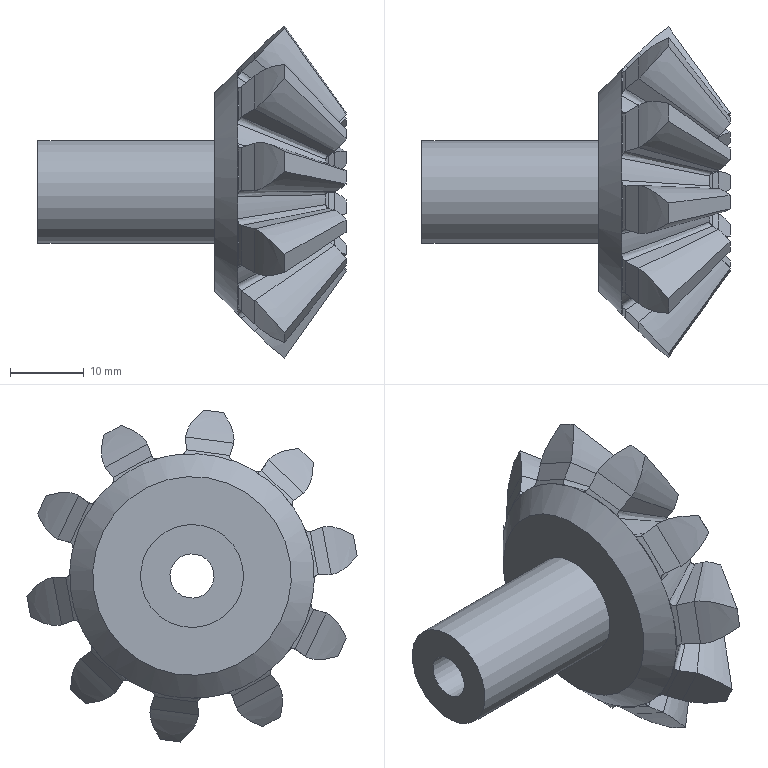Component | NX | BEVEL_GEAR_2 | 1 solid | 167 faces | volume 14449 mm3 | spline 100 | plane 43 | cone 22 | cylinder 2 | commonest cylinder face diameters 6 x1 14 x1